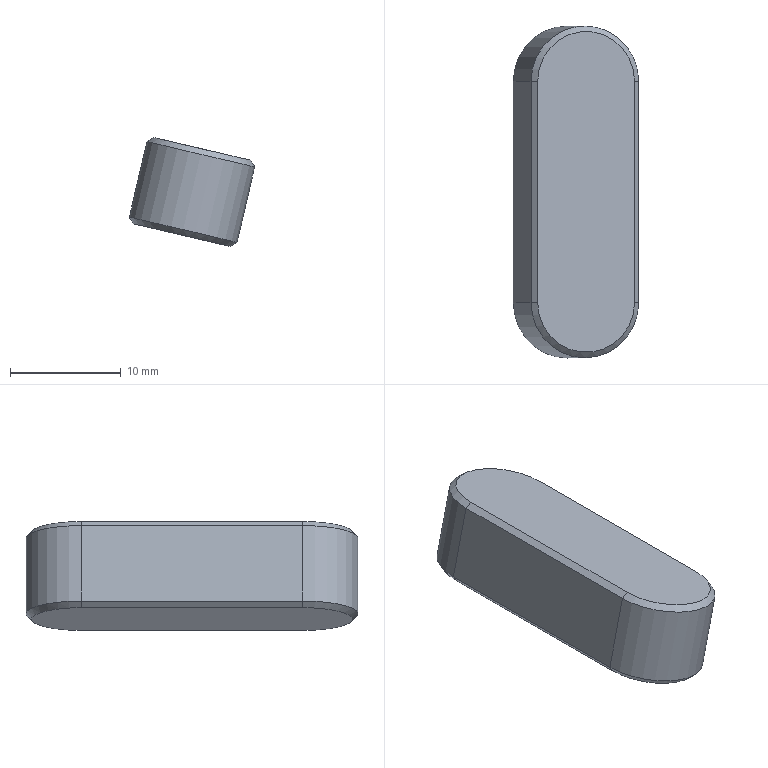Component | NX | SHAFT_KEY | 1 solid | 14 faces | box 11.34 x 30 x 9.85 mm | volume 2211 mm3 | plane 8 | cone 4 | cylinder 2 | commonest cylinder face diameters 10 x2
STEP:
#1=CARTESIAN_POINT('',(0.,0.,0.));
#2=DIRECTION('',(0.,0.,1.));
#3=DIRECTION('',(1.,0.,0.));
#4=AXIS2_PLACEMENT_3D('',#1,#2,#3);
#5=CARTESIAN_POINT('',(297.762,10.,102.339));
#6=VERTEX_POINT('',#5);
#7=CARTESIAN_POINT('',(299.362,10.,109.153));
#8=VERTEX_POINT('',#7);
#9=CARTESIAN_POINT('',(297.647,10.,101.852));
#10=DIRECTION('',(0.2286,0.,0.9735));
#11=VECTOR('',#10,1.);
#12=LINE('',#9,#11);
#13=CARTESIAN_POINT('',(302.515,10.,100.709));
#14=DIRECTION('',(0.2286,0.,0.9735));
#15=DIRECTION('',(0.,1.,0.));
#16=AXIS2_PLACEMENT_3D('',#13,#14,#15);
#17=CYLINDRICAL_SURFACE('',#16,5.);
#18=CARTESIAN_POINT('',(1.571,0.));
#19=DIRECTION('',(0.,1.));
#20=VECTOR('',#19,1.);
#21=LINE('',#18,#20);
#22=(GEOMETRIC_REPRESENTATION_CONTEXT(2)PARAMETRIC_REPRESENTATION_CONTEXT()REPRESENTATION_CONTEXT('',''));
#23=DEFINITIONAL_REPRESENTATION('',(#21),#22);
#24=PCURVE('',#17,#23);
#25=CARTESIAN_POINT('',(297.647,-10.,101.852));
#26=DIRECTION('',(0.9735,0.,-0.2286));
#27=DIRECTION('',(0.2286,0.,0.9735));
#28=AXIS2_PLACEMENT_3D('',#25,#26,#27);
#29=PLANE('',#28);
#30=CARTESIAN_POINT('',(0.,-20.));
#31=DIRECTION('',(1.,0.));
#32=VECTOR('',#31,1.);
#33=LINE('',#30,#32);
#34=(GEOMETRIC_REPRESENTATION_CONTEXT(2)PARAMETRIC_REPRESENTATION_CONTEXT()REPRESENTATION_CONTEXT('',''));
#35=DEFINITIONAL_REPRESENTATION('',(#33),#34);
#36=PCURVE('',#29,#35);
#37=SURFACE_CURVE('',#12,(#24,#36),.PCURVE_S1.);
#38=EDGE_CURVE('',#6,#8,#37,.T.);
#39=ORIENTED_EDGE('',*,*,#38,.T.);
#40=CARTESIAN_POINT('',(309.097,10.,106.867));
#41=VERTEX_POINT('',#40);
#42=CARTESIAN_POINT('',(304.229,10.,108.01));
#43=DIRECTION('',(-0.2286,0.,-0.9735));
#44=DIRECTION('',(0.,-1.,0.));
#45=AXIS2_PLACEMENT_3D('',#42,#43,#44);
#46=CIRCLE('',#45,5.);
#47=CARTESIAN_POINT('',(3.142,7.5));
#48=DIRECTION('',(-1.,0.));
#49=VECTOR('',#48,1.);
#50=LINE('',#47,#49);
#51=(GEOMETRIC_REPRESENTATION_CONTEXT(2)PARAMETRIC_REPRESENTATION_CONTEXT()REPRESENTATION_CONTEXT('',''));
#52=DEFINITIONAL_REPRESENTATION('',(#50),#51);
#53=PCURVE('',#17,#52);
#54=CARTESIAN_POINT('',(304.229,10.,108.01));
#55=DIRECTION('',(-0.2286,0.,-0.9735));
#56=DIRECTION('',(0.,-1.,-0.));
#57=AXIS2_PLACEMENT_3D('',#54,#55,#56);
#58=CONICAL_SURFACE('',#57,5.,0.7854);
#59=CARTESIAN_POINT('',(0.,0.));
#60=DIRECTION('',(1.,0.));
#61=VECTOR('',#60,1.);
#62=LINE('',#59,#61);
#63=(GEOMETRIC_REPRESENTATION_CONTEXT(2)PARAMETRIC_REPRESENTATION_CONTEXT()REPRESENTATION_CONTEXT('',''));
#64=DEFINITIONAL_REPRESENTATION('',(#62),#63);
#65=PCURVE('',#58,#64);
#66=SURFACE_CURVE('',#46,(#53,#65),.PCURVE_S1.);
#67=EDGE_CURVE('',#8,#41,#66,.T.);
#68=ORIENTED_EDGE('',*,*,#67,.T.);
#69=CARTESIAN_POINT('',(307.497,10.,100.052));
#70=VERTEX_POINT('',#69);
#71=CARTESIAN_POINT('',(307.382,10.,99.566));
#72=DIRECTION('',(0.2286,0.,0.9735));
#73=VECTOR('',#72,1.);
#74=LINE('',#71,#73);
#75=CARTESIAN_POINT('',(-1.571,-0.));
#76=DIRECTION('',(0.,1.));
#77=VECTOR('',#76,1.);
#78=LINE('',#75,#77);
#79=(GEOMETRIC_REPRESENTATION_CONTEXT(2)PARAMETRIC_REPRESENTATION_CONTEXT()REPRESENTATION_CONTEXT('',''));
#80=DEFINITIONAL_REPRESENTATION('',(#78),#79);
#81=PCURVE('',#17,#80);
#82=CARTESIAN_POINT('',(307.382,10.,99.566));
#83=DIRECTION('',(-0.9735,0.,0.2286));
#84=DIRECTION('',(-0.2286,0.,-0.9735));
#85=AXIS2_PLACEMENT_3D('',#82,#83,#84);
#86=PLANE('',#85);
#87=CARTESIAN_POINT('',(0.,0.));
#88=DIRECTION('',(-1.,0.));
#89=VECTOR('',#88,1.);
#90=LINE('',#87,#89);
#91=(GEOMETRIC_REPRESENTATION_CONTEXT(2)PARAMETRIC_REPRESENTATION_CONTEXT()REPRESENTATION_CONTEXT('',''));
#92=DEFINITIONAL_REPRESENTATION('',(#90),#91);
#93=PCURVE('',#86,#92);
#94=SURFACE_CURVE('',#74,(#81,#93),.PCURVE_S1.);
#95=EDGE_CURVE('',#70,#41,#94,.T.);
#96=ORIENTED_EDGE('',*,*,#95,.F.);
#97=CARTESIAN_POINT('',(302.629,10.,101.195));
#98=DIRECTION('',(0.2286,0.,0.9735));
#99=DIRECTION('',(0.,-1.,0.));
#100=AXIS2_PLACEMENT_3D('',#97,#98,#99);
#101=CIRCLE('',#100,5.);
#102=CARTESIAN_POINT('',(-3.142,0.5));
#103=DIRECTION('',(1.,0.));
#104=VECTOR('',#103,1.);
#105=LINE('',#102,#104);
#106=(GEOMETRIC_REPRESENTATION_CONTEXT(2)PARAMETRIC_REPRESENTATION_CONTEXT()REPRESENTATION_CONTEXT('',''));
#107=DEFINITIONAL_REPRESENTATION('',(#105),#106);
#108=PCURVE('',#17,#107);
#109=CARTESIAN_POINT('',(302.515,10.,100.709));
#110=DIRECTION('',(0.2286,0.,0.9735));
#111=DIRECTION('',(0.,1.,-0.));
#112=AXIS2_PLACEMENT_3D('',#109,#110,#111);
#113=CONICAL_SURFACE('',#112,4.5,0.7854);
#114=CARTESIAN_POINT('',(-3.142,0.5));
#115=DIRECTION('',(1.,0.));
#116=VECTOR('',#115,1.);
#117=LINE('',#114,#116);
#118=(GEOMETRIC_REPRESENTATION_CONTEXT(2)PARAMETRIC_REPRESENTATION_CONTEXT()REPRESENTATION_CONTEXT('',''));
#119=DEFINITIONAL_REPRESENTATION('',(#117),#118);
#120=PCURVE('',#113,#119);
#121=SURFACE_CURVE('',#101,(#108,#120),.PCURVE_S1.);
#122=EDGE_CURVE('',#70,#6,#121,.T.);
#123=ORIENTED_EDGE('',*,*,#122,.T.);
#124=EDGE_LOOP('',(#39,#68,#96,#123));
#125=FACE_BOUND('',#124,.T.);
#126=ADVANCED_FACE('',(#125),#17,.T.);
#127=ORIENTED_EDGE('',*,*,#95,.T.);
#128=CARTESIAN_POINT('',(309.097,-10.,106.867));
#129=VERTEX_POINT('',#128);
#130=CARTESIAN_POINT('',(309.097,10.,106.867));
#131=DIRECTION('',(0.,-1.,0.));
#132=VECTOR('',#131,1.);
#133=LINE('',#130,#132);
#134=CARTESIAN_POINT('',(-7.5,0.));
#135=DIRECTION('',(0.,1.));
#136=VECTOR('',#135,1.);
#137=LINE('',#134,#136);
#138=(GEOMETRIC_REPRESENTATION_CONTEXT(2)PARAMETRIC_REPRESENTATION_CONTEXT()REPRESENTATION_CONTEXT('',''));
#139=DEFINITIONAL_REPRESENTATION('',(#137),#138);
#140=PCURVE('',#86,#139);
#141=CARTESIAN_POINT('',(309.097,10.,106.867));
#142=DIRECTION('',(-0.85,0.,-0.5267));
#143=DIRECTION('',(0.,-1.,0.));
#144=AXIS2_PLACEMENT_3D('',#141,#142,#143);
#145=PLANE('',#144);
#146=CARTESIAN_POINT('',(0.,0.));
#147=DIRECTION('',(1.,0.));
#148=VECTOR('',#147,1.);
#149=LINE('',#146,#148);
#150=(GEOMETRIC_REPRESENTATION_CONTEXT(2)PARAMETRIC_REPRESENTATION_CONTEXT()REPRESENTATION_CONTEXT('',''));
#151=DEFINITIONAL_REPRESENTATION('',(#149),#150);
#152=PCURVE('',#145,#151);
#153=SURFACE_CURVE('',#133,(#140,#152),.PCURVE_S1.);
#154=EDGE_CURVE('',#41,#129,#153,.T.);
#155=ORIENTED_EDGE('',*,*,#154,.T.);
#156=CARTESIAN_POINT('',(307.497,-10.,100.052));
#157=VERTEX_POINT('',#156);
#158=CARTESIAN_POINT('',(307.382,-10.,99.566));
#159=DIRECTION('',(0.2286,0.,0.9735));
#160=VECTOR('',#159,1.);
#161=LINE('',#158,#160);
#162=CARTESIAN_POINT('',(0.,20.));
#163=DIRECTION('',(-1.,0.));
#164=VECTOR('',#163,1.);
#165=LINE('',#162,#164);
#166=(GEOMETRIC_REPRESENTATION_CONTEXT(2)PARAMETRIC_REPRESENTATION_CONTEXT()REPRESENTATION_CONTEXT('',''));
#167=DEFINITIONAL_REPRESENTATION('',(#165),#166);
#168=PCURVE('',#86,#167);
#169=CARTESIAN_POINT('',(302.515,-10.,100.709));
#170=DIRECTION('',(0.2286,0.,0.9735));
#171=DIRECTION('',(0.,1.,0.));
#172=AXIS2_PLACEMENT_3D('',#169,#170,#171);
#173=CYLINDRICAL_SURFACE('',#172,5.);
#174=CARTESIAN_POINT('',(4.712,-0.));
#175=DIRECTION('',(0.,1.));
#176=VECTOR('',#175,1.);
#177=LINE('',#174,#176);
#178=(GEOMETRIC_REPRESENTATION_CONTEXT(2)PARAMETRIC_REPRESENTATION_CONTEXT()REPRESENTATION_CONTEXT('',''));
#179=DEFINITIONAL_REPRESENTATION('',(#177),#178);
#180=PCURVE('',#173,#179);
#181=SURFACE_CURVE('',#161,(#168,#180),.PCURVE_S1.);
#182=EDGE_CURVE('',#157,#129,#181,.T.);
#183=ORIENTED_EDGE('',*,*,#182,.F.);
#184=CARTESIAN_POINT('',(307.497,10.,100.052));
#185=DIRECTION('',(0.,1.,0.));
#186=VECTOR('',#185,1.);
#187=LINE('',#184,#186);
#188=CARTESIAN_POINT('',(-0.5,0.));
#189=DIRECTION('',(0.,-1.));
#190=VECTOR('',#189,1.);
#191=LINE('',#188,#190);
#192=(GEOMETRIC_REPRESENTATION_CONTEXT(2)PARAMETRIC_REPRESENTATION_CONTEXT()REPRESENTATION_CONTEXT('',''));
#193=DEFINITIONAL_REPRESENTATION('',(#191),#192);
#194=PCURVE('',#86,#193);
#195=CARTESIAN_POINT('',(306.896,10.,99.68));
#196=DIRECTION('',(0.5267,0.,-0.85));
#197=DIRECTION('',(0.,1.,0.));
#198=AXIS2_PLACEMENT_3D('',#195,#196,#197);
#199=PLANE('',#198);
#200=CARTESIAN_POINT('',(-0.,0.7071));
#201=DIRECTION('',(1.,0.));
#202=VECTOR('',#201,1.);
#203=LINE('',#200,#202);
#204=(GEOMETRIC_REPRESENTATION_CONTEXT(2)PARAMETRIC_REPRESENTATION_CONTEXT()REPRESENTATION_CONTEXT('',''));
#205=DEFINITIONAL_REPRESENTATION('',(#203),#204);
#206=PCURVE('',#199,#205);
#207=SURFACE_CURVE('',#187,(#194,#206),.PCURVE_S1.);
#208=EDGE_CURVE('',#157,#70,#207,.T.);
#209=ORIENTED_EDGE('',*,*,#208,.T.);
#210=EDGE_LOOP('',(#127,#155,#183,#209));
#211=FACE_BOUND('',#210,.T.);
#212=ADVANCED_FACE('',(#211),#86,.F.);
#213=ORIENTED_EDGE('',*,*,#182,.T.);
#214=CARTESIAN_POINT('',(299.362,-10.,109.153));
#215=VERTEX_POINT('',#214);
#216=CARTESIAN_POINT('',(304.229,-10.,108.01));
#217=DIRECTION('',(-0.2286,0.,-0.9735));
#218=DIRECTION('',(0.,-1.,0.));
#219=AXIS2_PLACEMENT_3D('',#216,#217,#218);
#220=CIRCLE('',#219,5.);
#221=CARTESIAN_POINT('',(9.425,7.5));
#222=DIRECTION('',(-1.,0.));
#223=VECTOR('',#222,1.);
#224=LINE('',#221,#223);
#225=(GEOMETRIC_REPRESENTATION_CONTEXT(2)PARAMETRIC_REPRESENTATION_CONTEXT()REPRESENTATION_CONTEXT('',''));
#226=DEFINITIONAL_REPRESENTATION('',(#224),#225);
#227=PCURVE('',#173,#226);
#228=CARTESIAN_POINT('',(304.229,-10.,108.01));
#229=DIRECTION('',(-0.2286,0.,-0.9735));
#230=DIRECTION('',(0.,-1.,-0.));
#231=AXIS2_PLACEMENT_3D('',#228,#229,#230);
#232=CONICAL_SURFACE('',#231,5.,0.7854);
#233=CARTESIAN_POINT('',(0.,0.));
#234=DIRECTION('',(1.,0.));
#235=VECTOR('',#234,1.);
#236=LINE('',#233,#235);
#237=(GEOMETRIC_REPRESENTATION_CONTEXT(2)PARAMETRIC_REPRESENTATION_CONTEXT()REPRESENTATION_CONTEXT('',''));
#238=DEFINITIONAL_REPRESENTATION('',(#236),#237);
#239=PCURVE('',#232,#238);
#240=SURFACE_CURVE('',#220,(#227,#239),.PCURVE_S1.);
#241=EDGE_CURVE('',#129,#215,#240,.T.);
#242=ORIENTED_EDGE('',*,*,#241,.T.);
#243=CARTESIAN_POINT('',(297.762,-10.,102.339));
#244=VERTEX_POINT('',#243);
#245=CARTESIAN_POINT('',(297.647,-10.,101.852));
#246=DIRECTION('',(0.2286,0.,0.9735));
#247=VECTOR('',#246,1.);
#248=LINE('',#245,#247);
#249=CARTESIAN_POINT('',(1.571,0.));
#250=DIRECTION('',(0.,1.));
#251=VECTOR('',#250,1.);
#252=LINE('',#249,#251);
#253=(GEOMETRIC_REPRESENTATION_CONTEXT(2)PARAMETRIC_REPRESENTATION_CONTEXT()REPRESENTATION_CONTEXT('',''));
#254=DEFINITIONAL_REPRESENTATION('',(#252),#253);
#255=PCURVE('',#173,#254);
#256=CARTESIAN_POINT('',(0.,0.));
#257=DIRECTION('',(1.,0.));
#258=VECTOR('',#257,1.);
#259=LINE('',#256,#258);
#260=(GEOMETRIC_REPRESENTATION_CONTEXT(2)PARAMETRIC_REPRESENTATION_CONTEXT()REPRESENTATION_CONTEXT('',''));
#261=DEFINITIONAL_REPRESENTATION('',(#259),#260);
#262=PCURVE('',#29,#261);
#263=SURFACE_CURVE('',#248,(#255,#262),.PCURVE_S1.);
#264=EDGE_CURVE('',#244,#215,#263,.T.);
#265=ORIENTED_EDGE('',*,*,#264,.F.);
#266=CARTESIAN_POINT('',(302.629,-10.,101.195));
#267=DIRECTION('',(0.2286,0.,0.9735));
#268=DIRECTION('',(0.,-1.,0.));
#269=AXIS2_PLACEMENT_3D('',#266,#267,#268);
#270=CIRCLE('',#269,5.);
#271=CARTESIAN_POINT('',(-3.142,0.5));
#272=DIRECTION('',(1.,0.));
#273=VECTOR('',#272,1.);
#274=LINE('',#271,#273);
#275=(GEOMETRIC_REPRESENTATION_CONTEXT(2)PARAMETRIC_REPRESENTATION_CONTEXT()REPRESENTATION_CONTEXT('',''));
#276=DEFINITIONAL_REPRESENTATION('',(#274),#275);
#277=PCURVE('',#173,#276);
#278=CARTESIAN_POINT('',(302.515,-10.,100.709));
#279=DIRECTION('',(0.2286,0.,0.9735));
#280=DIRECTION('',(0.,1.,-0.));
#281=AXIS2_PLACEMENT_3D('',#278,#279,#280);
#282=CONICAL_SURFACE('',#281,4.5,0.7854);
#283=CARTESIAN_POINT('',(-3.142,0.5));
#284=DIRECTION('',(1.,-0.));
#285=VECTOR('',#284,1.);
#286=LINE('',#283,#285);
#287=(GEOMETRIC_REPRESENTATION_CONTEXT(2)PARAMETRIC_REPRESENTATION_CONTEXT()REPRESENTATION_CONTEXT('',''));
#288=DEFINITIONAL_REPRESENTATION('',(#286),#287);
#289=PCURVE('',#282,#288);
#290=SURFACE_CURVE('',#270,(#277,#289),.PCURVE_S1.);
#291=EDGE_CURVE('',#244,#157,#290,.T.);
#292=ORIENTED_EDGE('',*,*,#291,.T.);
#293=EDGE_LOOP('',(#213,#242,#265,#292));
#294=FACE_BOUND('',#293,.T.);
#295=ADVANCED_FACE('',(#294),#173,.T.);
#296=ORIENTED_EDGE('',*,*,#264,.T.);
#297=CARTESIAN_POINT('',(299.362,-10.,109.153));
#298=DIRECTION('',(0.,1.,0.));
#299=VECTOR('',#298,1.);
#300=LINE('',#297,#299);
#301=CARTESIAN_POINT('',(7.5,0.));
#302=DIRECTION('',(0.,-1.));
#303=VECTOR('',#302,1.);
#304=LINE('',#301,#303);
#305=(GEOMETRIC_REPRESENTATION_CONTEXT(2)PARAMETRIC_REPRESENTATION_CONTEXT()REPRESENTATION_CONTEXT('',''));
#306=DEFINITIONAL_REPRESENTATION('',(#304),#305);
#307=PCURVE('',#29,#306);
#308=CARTESIAN_POINT('',(299.362,-10.,109.153));
#309=DIRECTION('',(0.5267,0.,-0.85));
#310=DIRECTION('',(0.,1.,0.));
#311=AXIS2_PLACEMENT_3D('',#308,#309,#310);
#312=PLANE('',#311);
#313=CARTESIAN_POINT('',(0.,0.));
#314=DIRECTION('',(1.,0.));
#315=VECTOR('',#314,1.);
#316=LINE('',#313,#315);
#317=(GEOMETRIC_REPRESENTATION_CONTEXT(2)PARAMETRIC_REPRESENTATION_CONTEXT()REPRESENTATION_CONTEXT('',''));
#318=DEFINITIONAL_REPRESENTATION('',(#316),#317);
#319=PCURVE('',#312,#318);
#320=SURFACE_CURVE('',#300,(#307,#319),.PCURVE_S1.);
#321=EDGE_CURVE('',#215,#8,#320,.T.);
#322=ORIENTED_EDGE('',*,*,#321,.T.);
#323=ORIENTED_EDGE('',*,*,#38,.F.);
#324=CARTESIAN_POINT('',(297.762,-10.,102.339));
#325=DIRECTION('',(0.,-1.,0.));
#326=VECTOR('',#325,1.);
#327=LINE('',#324,#326);
#328=CARTESIAN_POINT('',(0.5,0.));
#329=DIRECTION('',(0.,1.));
#330=VECTOR('',#329,1.);
#331=LINE('',#328,#330);
#332=(GEOMETRIC_REPRESENTATION_CONTEXT(2)PARAMETRIC_REPRESENTATION_CONTEXT()REPRESENTATION_CONTEXT('',''));
#333=DEFINITIONAL_REPRESENTATION('',(#331),#332);
#334=PCURVE('',#29,#333);
#335=CARTESIAN_POINT('',(298.134,10.,101.737));
#336=DIRECTION('',(-0.85,0.,-0.5267));
#337=DIRECTION('',(0.,-1.,0.));
#338=AXIS2_PLACEMENT_3D('',#335,#336,#337);
#339=PLANE('',#338);
#340=CARTESIAN_POINT('',(20.,0.7071));
#341=DIRECTION('',(1.,0.));
#342=VECTOR('',#341,1.);
#343=LINE('',#340,#342);
#344=(GEOMETRIC_REPRESENTATION_CONTEXT(2)PARAMETRIC_REPRESENTATION_CONTEXT()REPRESENTATION_CONTEXT('',''));
#345=DEFINITIONAL_REPRESENTATION('',(#343),#344);
#346=PCURVE('',#339,#345);
#347=SURFACE_CURVE('',#327,(#334,#346),.PCURVE_S1.);
#348=EDGE_CURVE('',#6,#244,#347,.T.);
#349=ORIENTED_EDGE('',*,*,#348,.T.);
#350=EDGE_LOOP('',(#296,#322,#323,#349));
#351=FACE_BOUND('',#350,.T.);
#352=ADVANCED_FACE('',(#351),#29,.F.);
#353=CARTESIAN_POINT('',(298.134,-10.,101.737));
#354=VERTEX_POINT('',#353);
#355=CARTESIAN_POINT('',(298.134,10.,101.737));
#356=VERTEX_POINT('',#355);
#357=CARTESIAN_POINT('',(298.134,10.,101.737));
#358=DIRECTION('',(0.,1.,0.));
#359=VECTOR('',#358,1.);
#360=LINE('',#357,#359);
#361=CARTESIAN_POINT('',(302.515,10.,100.709));
#362=DIRECTION('',(-0.2286,0.,-0.9735));
#363=DIRECTION('',(0.,-1.,0.));
#364=AXIS2_PLACEMENT_3D('',#361,#362,#363);
#365=PLANE('',#364);
#366=CARTESIAN_POINT('',(0.,4.5));
#367=DIRECTION('',(-1.,0.));
#368=VECTOR('',#367,1.);
#369=LINE('',#366,#368);
#370=(GEOMETRIC_REPRESENTATION_CONTEXT(2)PARAMETRIC_REPRESENTATION_CONTEXT()REPRESENTATION_CONTEXT('',''));
#371=DEFINITIONAL_REPRESENTATION('',(#369),#370);
#372=PCURVE('',#365,#371);
#373=CARTESIAN_POINT('',(0.,0.));
#374=DIRECTION('',(-1.,0.));
#375=VECTOR('',#374,1.);
#376=LINE('',#373,#375);
#377=(GEOMETRIC_REPRESENTATION_CONTEXT(2)PARAMETRIC_REPRESENTATION_CONTEXT()REPRESENTATION_CONTEXT('',''));
#378=DEFINITIONAL_REPRESENTATION('',(#376),#377);
#379=PCURVE('',#339,#378);
#380=SURFACE_CURVE('',#360,(#372,#379),.PCURVE_S1.);
#381=EDGE_CURVE('',#354,#356,#380,.T.);
#382=ORIENTED_EDGE('',*,*,#381,.T.);
#383=CARTESIAN_POINT('',(306.896,10.,99.68));
#384=VERTEX_POINT('',#383);
#385=CARTESIAN_POINT('',(302.515,10.,100.709));
#386=DIRECTION('',(-0.2286,0.,-0.9735));
#387=DIRECTION('',(0.,-1.,0.));
#388=AXIS2_PLACEMENT_3D('',#385,#386,#387);
#389=CIRCLE('',#388,4.5);
#390=CARTESIAN_POINT('',(0.,0.));
#391=DIRECTION('',(1.,0.));
#392=AXIS2_PLACEMENT_2D('',#390,#391);
#393=CIRCLE('',#392,4.5);
#394=(GEOMETRIC_REPRESENTATION_CONTEXT(2)PARAMETRIC_REPRESENTATION_CONTEXT()REPRESENTATION_CONTEXT('',''));
#395=DEFINITIONAL_REPRESENTATION('',(#393),#394);
#396=PCURVE('',#365,#395);
#397=CARTESIAN_POINT('',(3.142,0.));
#398=DIRECTION('',(-1.,-0.));
#399=VECTOR('',#398,1.);
#400=LINE('',#397,#399);
#401=(GEOMETRIC_REPRESENTATION_CONTEXT(2)PARAMETRIC_REPRESENTATION_CONTEXT()REPRESENTATION_CONTEXT('',''));
#402=DEFINITIONAL_REPRESENTATION('',(#400),#401);
#403=PCURVE('',#113,#402);
#404=SURFACE_CURVE('',#389,(#396,#403),.PCURVE_S1.);
#405=EDGE_CURVE('',#356,#384,#404,.T.);
#406=ORIENTED_EDGE('',*,*,#405,.T.);
#407=CARTESIAN_POINT('',(306.896,-10.,99.68));
#408=VERTEX_POINT('',#407);
#409=CARTESIAN_POINT('',(306.896,-10.,99.68));
#410=DIRECTION('',(0.,-1.,0.));
#411=VECTOR('',#410,1.);
#412=LINE('',#409,#411);
#413=CARTESIAN_POINT('',(20.,-4.5));
#414=DIRECTION('',(1.,0.));
#415=VECTOR('',#414,1.);
#416=LINE('',#413,#415);
#417=(GEOMETRIC_REPRESENTATION_CONTEXT(2)PARAMETRIC_REPRESENTATION_CONTEXT()REPRESENTATION_CONTEXT('',''));
#418=DEFINITIONAL_REPRESENTATION('',(#416),#417);
#419=PCURVE('',#365,#418);
#420=CARTESIAN_POINT('',(-20.,0.));
#421=DIRECTION('',(-1.,0.));
#422=VECTOR('',#421,1.);
#423=LINE('',#420,#422);
#424=(GEOMETRIC_REPRESENTATION_CONTEXT(2)PARAMETRIC_REPRESENTATION_CONTEXT()REPRESENTATION_CONTEXT('',''));
#425=DEFINITIONAL_REPRESENTATION('',(#423),#424);
#426=PCURVE('',#199,#425);
#427=SURFACE_CURVE('',#412,(#419,#426),.PCURVE_S1.);
#428=EDGE_CURVE('',#384,#408,#427,.T.);
#429=ORIENTED_EDGE('',*,*,#428,.T.);
#430=CARTESIAN_POINT('',(302.515,-10.,100.709));
#431=DIRECTION('',(-0.2286,0.,-0.9735));
#432=DIRECTION('',(0.,-1.,0.));
#433=AXIS2_PLACEMENT_3D('',#430,#431,#432);
#434=CIRCLE('',#433,4.5);
#435=CARTESIAN_POINT('',(20.,0.));
#436=DIRECTION('',(1.,0.));
#437=AXIS2_PLACEMENT_2D('',#435,#436);
#438=CIRCLE('',#437,4.5);
#439=(GEOMETRIC_REPRESENTATION_CONTEXT(2)PARAMETRIC_REPRESENTATION_CONTEXT()REPRESENTATION_CONTEXT('',''));
#440=DEFINITIONAL_REPRESENTATION('',(#438),#439);
#441=PCURVE('',#365,#440);
#442=CARTESIAN_POINT('',(9.425,-0.));
#443=DIRECTION('',(-1.,0.));
#444=VECTOR('',#443,1.);
#445=LINE('',#442,#444);
#446=(GEOMETRIC_REPRESENTATION_CONTEXT(2)PARAMETRIC_REPRESENTATION_CONTEXT()REPRESENTATION_CONTEXT('',''));
#447=DEFINITIONAL_REPRESENTATION('',(#445),#446);
#448=PCURVE('',#282,#447);
#449=SURFACE_CURVE('',#434,(#441,#448),.PCURVE_S1.);
#450=EDGE_CURVE('',#408,#354,#449,.T.);
#451=ORIENTED_EDGE('',*,*,#450,.T.);
#452=EDGE_LOOP('',(#382,#406,#429,#451));
#453=FACE_BOUND('',#452,.T.);
#454=ADVANCED_FACE('',(#453),#365,.T.);
#455=CARTESIAN_POINT('',(308.725,-10.,107.468));
#456=VERTEX_POINT('',#455);
#457=CARTESIAN_POINT('',(308.725,10.,107.468));
#458=VERTEX_POINT('',#457);
#459=CARTESIAN_POINT('',(308.725,10.,107.468));
#460=DIRECTION('',(0.,1.,0.));
#461=VECTOR('',#460,1.);
#462=LINE('',#459,#461);
#463=CARTESIAN_POINT('',(304.344,10.,108.497));
#464=DIRECTION('',(-0.2286,0.,-0.9735));
#465=DIRECTION('',(0.,-1.,0.));
#466=AXIS2_PLACEMENT_3D('',#463,#464,#465);
#467=PLANE('',#466);
#468=CARTESIAN_POINT('',(0.,-4.5));
#469=DIRECTION('',(-1.,0.));
#470=VECTOR('',#469,1.);
#471=LINE('',#468,#470);
#472=(GEOMETRIC_REPRESENTATION_CONTEXT(2)PARAMETRIC_REPRESENTATION_CONTEXT()REPRESENTATION_CONTEXT('',''));
#473=DEFINITIONAL_REPRESENTATION('',(#471),#472);
#474=PCURVE('',#467,#473);
#475=CARTESIAN_POINT('',(0.,0.7071));
#476=DIRECTION('',(-1.,0.));
#477=VECTOR('',#476,1.);
#478=LINE('',#475,#477);
#479=(GEOMETRIC_REPRESENTATION_CONTEXT(2)PARAMETRIC_REPRESENTATION_CONTEXT()REPRESENTATION_CONTEXT('',''));
#480=DEFINITIONAL_REPRESENTATION('',(#478),#479);
#481=PCURVE('',#145,#480);
#482=SURFACE_CURVE('',#462,(#474,#481),.PCURVE_S1.);
#483=EDGE_CURVE('',#456,#458,#482,.T.);
#484=ORIENTED_EDGE('',*,*,#483,.T.);
#485=CARTESIAN_POINT('',(299.963,10.,109.526));
#486=VERTEX_POINT('',#485);
#487=CARTESIAN_POINT('',(304.344,10.,108.497));
#488=DIRECTION('',(0.2286,0.,0.9735));
#489=DIRECTION('',(0.,-1.,0.));
#490=AXIS2_PLACEMENT_3D('',#487,#488,#489);
#491=CIRCLE('',#490,4.5);
#492=CARTESIAN_POINT('',(4.5,0.));
#493=CARTESIAN_POINT('',(4.5,-7.794));
#494=CARTESIAN_POINT('',(-2.25,-3.897));
#495=CARTESIAN_POINT('',(-9.,-0.));
#496=CARTESIAN_POINT('',(-2.25,3.897));
#497=CARTESIAN_POINT('',(4.5,7.794));
#498=CARTESIAN_POINT('',(4.5,0.));
#499=(BOUNDED_CURVE()B_SPLINE_CURVE(2,(#492,#493,#494,#495,#496,#497,#498),.UNSPECIFIED.,.T.,.F.)B_SPLINE_CURVE_WITH_KNOTS((1,2,2,2,2,1),(-2.094,0.,2.094,4.189,6.283,8.378),.UNSPECIFIED.)CURVE()GEOMETRIC_REPRESENTATION_ITEM()RATIONAL_B_SPLINE_CURVE((1.,0.5,1.,0.5,1.,0.5,1.))REPRESENTATION_ITEM(''));
#500=(GEOMETRIC_REPRESENTATION_CONTEXT(2)PARAMETRIC_REPRESENTATION_CONTEXT()REPRESENTATION_CONTEXT('',''));
#501=DEFINITIONAL_REPRESENTATION('',(#499),#500);
#502=PCURVE('',#467,#501);
#503=CARTESIAN_POINT('',(6.283,-0.5));
#504=DIRECTION('',(-1.,-0.));
#505=VECTOR('',#504,1.);
#506=LINE('',#503,#505);
#507=(GEOMETRIC_REPRESENTATION_CONTEXT(2)PARAMETRIC_REPRESENTATION_CONTEXT()REPRESENTATION_CONTEXT('',''));
#508=DEFINITIONAL_REPRESENTATION('',(#506),#507);
#509=PCURVE('',#58,#508);
#510=SURFACE_CURVE('',#491,(#502,#509),.PCURVE_S1.);
#511=EDGE_CURVE('',#458,#486,#510,.T.);
#512=ORIENTED_EDGE('',*,*,#511,.T.);
#513=CARTESIAN_POINT('',(299.963,-10.,109.526));
#514=VERTEX_POINT('',#513);
#515=CARTESIAN_POINT('',(299.963,10.,109.526));
#516=DIRECTION('',(0.,-1.,0.));
#517=VECTOR('',#516,1.);
#518=LINE('',#515,#517);
#519=CARTESIAN_POINT('',(0.,4.5));
#520=DIRECTION('',(1.,0.));
#521=VECTOR('',#520,1.);
#522=LINE('',#519,#521);
#523=(GEOMETRIC_REPRESENTATION_CONTEXT(2)PARAMETRIC_REPRESENTATION_CONTEXT()REPRESENTATION_CONTEXT('',''));
#524=DEFINITIONAL_REPRESENTATION('',(#522),#523);
#525=PCURVE('',#467,#524);
#526=CARTESIAN_POINT('',(20.,0.7071));
#527=DIRECTION('',(-1.,0.));
#528=VECTOR('',#527,1.);
#529=LINE('',#526,#528);
#530=(GEOMETRIC_REPRESENTATION_CONTEXT(2)PARAMETRIC_REPRESENTATION_CONTEXT()REPRESENTATION_CONTEXT('',''));
#531=DEFINITIONAL_REPRESENTATION('',(#529),#530);
#532=PCURVE('',#312,#531);
#533=SURFACE_CURVE('',#518,(#525,#532),.PCURVE_S1.);
#534=EDGE_CURVE('',#486,#514,#533,.T.);
#535=ORIENTED_EDGE('',*,*,#534,.T.);
#536=CARTESIAN_POINT('',(304.344,-10.,108.497));
#537=DIRECTION('',(0.2286,0.,0.9735));
#538=DIRECTION('',(0.,-1.,0.));
#539=AXIS2_PLACEMENT_3D('',#536,#537,#538);
#540=CIRCLE('',#539,4.5);
#541=CARTESIAN_POINT('',(24.5,0.));
#542=CARTESIAN_POINT('',(24.5,-7.794));
#543=CARTESIAN_POINT('',(17.75,-3.897));
#544=CARTESIAN_POINT('',(11.,-0.));
#545=CARTESIAN_POINT('',(17.75,3.897));
#546=CARTESIAN_POINT('',(24.5,7.794));
#547=CARTESIAN_POINT('',(24.5,0.));
#548=(BOUNDED_CURVE()B_SPLINE_CURVE(2,(#541,#542,#543,#544,#545,#546,#547),.UNSPECIFIED.,.T.,.F.)B_SPLINE_CURVE_WITH_KNOTS((1,2,2,2,2,1),(-2.094,0.,2.094,4.189,6.283,8.378),.UNSPECIFIED.)CURVE()GEOMETRIC_REPRESENTATION_ITEM()RATIONAL_B_SPLINE_CURVE((1.,0.5,1.,0.5,1.,0.5,1.))REPRESENTATION_ITEM(''));
#549=(GEOMETRIC_REPRESENTATION_CONTEXT(2)PARAMETRIC_REPRESENTATION_CONTEXT()REPRESENTATION_CONTEXT('',''));
#550=DEFINITIONAL_REPRESENTATION('',(#548),#549);
#551=PCURVE('',#467,#550);
#552=CARTESIAN_POINT('',(12.566,-0.5));
#553=DIRECTION('',(-1.,0.));
#554=VECTOR('',#553,1.);
#555=LINE('',#552,#554);
#556=(GEOMETRIC_REPRESENTATION_CONTEXT(2)PARAMETRIC_REPRESENTATION_CONTEXT()REPRESENTATION_CONTEXT('',''));
#557=DEFINITIONAL_REPRESENTATION('',(#555),#556);
#558=PCURVE('',#232,#557);
#559=SURFACE_CURVE('',#540,(#551,#558),.PCURVE_S1.);
#560=EDGE_CURVE('',#514,#456,#559,.T.);
#561=ORIENTED_EDGE('',*,*,#560,.T.);
#562=EDGE_LOOP('',(#484,#512,#535,#561));
#563=FACE_BOUND('',#562,.T.);
#564=ADVANCED_FACE('',(#563),#467,.F.);
#565=CARTESIAN_POINT('',(308.725,-10.,107.468));
#566=DIRECTION('',(0.5267,0.,-0.85));
#567=VECTOR('',#566,1.);
#568=LINE('',#565,#567);
#569=CARTESIAN_POINT('',(4.712,-0.5));
#570=DIRECTION('',(0.,1.));
#571=VECTOR('',#570,1.);
#572=LINE('',#569,#571);
#573=(GEOMETRIC_REPRESENTATION_CONTEXT(2)PARAMETRIC_REPRESENTATION_CONTEXT()REPRESENTATION_CONTEXT('',''));
#574=DEFINITIONAL_REPRESENTATION('',(#572),#573);
#575=PCURVE('',#232,#574);
#576=CARTESIAN_POINT('',(20.,0.7071));
#577=DIRECTION('',(0.,-1.));
#578=VECTOR('',#577,1.);
#579=LINE('',#576,#578);
#580=(GEOMETRIC_REPRESENTATION_CONTEXT(2)PARAMETRIC_REPRESENTATION_CONTEXT()REPRESENTATION_CONTEXT('',''));
#581=DEFINITIONAL_REPRESENTATION('',(#579),#580);
#582=PCURVE('',#145,#581);
#583=SURFACE_CURVE('',#568,(#575,#582),.PCURVE_S1.);
#584=EDGE_CURVE('',#456,#129,#583,.T.);
#585=ORIENTED_EDGE('',*,*,#584,.F.);
#586=ORIENTED_EDGE('',*,*,#560,.F.);
#587=CARTESIAN_POINT('',(299.362,-10.,109.153));
#588=DIRECTION('',(0.85,0.,0.5267));
#589=VECTOR('',#588,1.);
#590=LINE('',#587,#589);
#591=CARTESIAN_POINT('',(7.854,-0.));
#592=DIRECTION('',(-0.,-1.));
#593=VECTOR('',#592,1.);
#594=LINE('',#591,#593);
#595=(GEOMETRIC_REPRESENTATION_CONTEXT(2)PARAMETRIC_REPRESENTATION_CONTEXT()REPRESENTATION_CONTEXT('',''));
#596=DEFINITIONAL_REPRESENTATION('',(#594),#595);
#597=PCURVE('',#232,#596);
#598=CARTESIAN_POINT('',(-0.,0.));
#599=DIRECTION('',(0.,1.));
#600=VECTOR('',#599,1.);
#601=LINE('',#598,#600);
#602=(GEOMETRIC_REPRESENTATION_CONTEXT(2)PARAMETRIC_REPRESENTATION_CONTEXT()REPRESENTATION_CONTEXT('',''));
#603=DEFINITIONAL_REPRESENTATION('',(#601),#602);
#604=PCURVE('',#312,#603);
#605=SURFACE_CURVE('',#590,(#597,#604),.PCURVE_S1.);
#606=EDGE_CURVE('',#215,#514,#605,.T.);
#607=ORIENTED_EDGE('',*,*,#606,.F.);
#608=ORIENTED_EDGE('',*,*,#241,.F.);
#609=EDGE_LOOP('',(#585,#586,#607,#608));
#610=FACE_BOUND('',#609,.T.);
#611=ADVANCED_FACE('',(#610),#232,.T.);
#612=ORIENTED_EDGE('',*,*,#606,.T.);
#613=ORIENTED_EDGE('',*,*,#534,.F.);
#614=CARTESIAN_POINT('',(299.362,10.,109.153));
#615=DIRECTION('',(0.85,0.,0.5267));
#616=VECTOR('',#615,1.);
#617=LINE('',#614,#616);
#618=CARTESIAN_POINT('',(20.,0.));
#619=DIRECTION('',(0.,1.));
#620=VECTOR('',#619,1.);
#621=LINE('',#618,#620);
#622=(GEOMETRIC_REPRESENTATION_CONTEXT(2)PARAMETRIC_REPRESENTATION_CONTEXT()REPRESENTATION_CONTEXT('',''));
#623=DEFINITIONAL_REPRESENTATION('',(#621),#622);
#624=PCURVE('',#312,#623);
#625=CARTESIAN_POINT('',(1.571,-0.));
#626=DIRECTION('',(0.,-1.));
#627=VECTOR('',#626,1.);
#628=LINE('',#625,#627);
#629=(GEOMETRIC_REPRESENTATION_CONTEXT(2)PARAMETRIC_REPRESENTATION_CONTEXT()REPRESENTATION_CONTEXT('',''));
#630=DEFINITIONAL_REPRESENTATION('',(#628),#629);
#631=PCURVE('',#58,#630);
#632=SURFACE_CURVE('',#617,(#624,#631),.PCURVE_S1.);
#633=EDGE_CURVE('',#8,#486,#632,.T.);
#634=ORIENTED_EDGE('',*,*,#633,.F.);
#635=ORIENTED_EDGE('',*,*,#321,.F.);
#636=EDGE_LOOP('',(#612,#613,#634,#635));
#637=FACE_BOUND('',#636,.T.);
#638=ADVANCED_FACE('',(#637),#312,.F.);
#639=ORIENTED_EDGE('',*,*,#584,.T.);
#640=ORIENTED_EDGE('',*,*,#154,.F.);
#641=CARTESIAN_POINT('',(308.725,10.,107.468));
#642=DIRECTION('',(0.5267,-0.,-0.85));
#643=VECTOR('',#642,1.);
#644=LINE('',#641,#643);
#645=CARTESIAN_POINT('',(0.,0.7071));
#646=DIRECTION('',(0.,-1.));
#647=VECTOR('',#646,1.);
#648=LINE('',#645,#647);
#649=(GEOMETRIC_REPRESENTATION_CONTEXT(2)PARAMETRIC_REPRESENTATION_CONTEXT()REPRESENTATION_CONTEXT('',''));
#650=DEFINITIONAL_REPRESENTATION('',(#648),#649);
#651=PCURVE('',#145,#650);
#652=CARTESIAN_POINT('',(4.712,-0.5));
#653=DIRECTION('',(0.,1.));
#654=VECTOR('',#653,1.);
#655=LINE('',#652,#654);
#656=(GEOMETRIC_REPRESENTATION_CONTEXT(2)PARAMETRIC_REPRESENTATION_CONTEXT()REPRESENTATION_CONTEXT('',''));
#657=DEFINITIONAL_REPRESENTATION('',(#655),#656);
#658=PCURVE('',#58,#657);
#659=SURFACE_CURVE('',#644,(#651,#658),.PCURVE_S1.);
#660=EDGE_CURVE('',#458,#41,#659,.T.);
#661=ORIENTED_EDGE('',*,*,#660,.F.);
#662=ORIENTED_EDGE('',*,*,#483,.F.);
#663=EDGE_LOOP('',(#639,#640,#661,#662));
#664=FACE_BOUND('',#663,.T.);
#665=ADVANCED_FACE('',(#664),#145,.F.);
#666=ORIENTED_EDGE('',*,*,#633,.T.);
#667=ORIENTED_EDGE('',*,*,#511,.F.);
#668=ORIENTED_EDGE('',*,*,#660,.T.);
#669=ORIENTED_EDGE('',*,*,#67,.F.);
#670=EDGE_LOOP('',(#666,#667,#668,#669));
#671=FACE_BOUND('',#670,.T.);
#672=ADVANCED_FACE('',(#671),#58,.T.);
#673=CARTESIAN_POINT('',(307.497,-10.,100.052));
#674=DIRECTION('',(-0.85,0.,-0.5267));
#675=VECTOR('',#674,1.);
#676=LINE('',#673,#675);
#677=CARTESIAN_POINT('',(4.712,0.5));
#678=DIRECTION('',(0.,-1.));
#679=VECTOR('',#678,1.);
#680=LINE('',#677,#679);
#681=(GEOMETRIC_REPRESENTATION_CONTEXT(2)PARAMETRIC_REPRESENTATION_CONTEXT()REPRESENTATION_CONTEXT('',''));
#682=DEFINITIONAL_REPRESENTATION('',(#680),#681);
#683=PCURVE('',#282,#682);
#684=CARTESIAN_POINT('',(-20.,0.7071));
#685=DIRECTION('',(0.,-1.));
#686=VECTOR('',#685,1.);
#687=LINE('',#684,#686);
#688=(GEOMETRIC_REPRESENTATION_CONTEXT(2)PARAMETRIC_REPRESENTATION_CONTEXT()REPRESENTATION_CONTEXT('',''));
#689=DEFINITIONAL_REPRESENTATION('',(#687),#688);
#690=PCURVE('',#199,#689);
#691=SURFACE_CURVE('',#676,(#683,#690),.PCURVE_S1.);
#692=EDGE_CURVE('',#157,#408,#691,.T.);
#693=ORIENTED_EDGE('',*,*,#692,.F.);
#694=ORIENTED_EDGE('',*,*,#291,.F.);
#695=CARTESIAN_POINT('',(298.134,-10.,101.737));
#696=DIRECTION('',(-0.5267,0.,0.85));
#697=VECTOR('',#696,1.);
#698=LINE('',#695,#697);
#699=CARTESIAN_POINT('',(1.571,-0.));
#700=DIRECTION('',(-0.,1.));
#701=VECTOR('',#700,1.);
#702=LINE('',#699,#701);
#703=(GEOMETRIC_REPRESENTATION_CONTEXT(2)PARAMETRIC_REPRESENTATION_CONTEXT()REPRESENTATION_CONTEXT('',''));
#704=DEFINITIONAL_REPRESENTATION('',(#702),#703);
#705=PCURVE('',#282,#704);
#706=CARTESIAN_POINT('',(20.,0.));
#707=DIRECTION('',(0.,1.));
#708=VECTOR('',#707,1.);
#709=LINE('',#706,#708);
#710=(GEOMETRIC_REPRESENTATION_CONTEXT(2)PARAMETRIC_REPRESENTATION_CONTEXT()REPRESENTATION_CONTEXT('',''));
#711=DEFINITIONAL_REPRESENTATION('',(#709),#710);
#712=PCURVE('',#339,#711);
#713=SURFACE_CURVE('',#698,(#705,#712),.PCURVE_S1.);
#714=EDGE_CURVE('',#354,#244,#713,.T.);
#715=ORIENTED_EDGE('',*,*,#714,.F.);
#716=ORIENTED_EDGE('',*,*,#450,.F.);
#717=EDGE_LOOP('',(#693,#694,#715,#716));
#718=FACE_BOUND('',#717,.T.);
#719=ADVANCED_FACE('',(#718),#282,.T.);
#720=ORIENTED_EDGE('',*,*,#714,.T.);
#721=ORIENTED_EDGE('',*,*,#348,.F.);
#722=CARTESIAN_POINT('',(298.134,10.,101.737));
#723=DIRECTION('',(-0.5267,-0.,0.85));
#724=VECTOR('',#723,1.);
#725=LINE('',#722,#724);
#726=CARTESIAN_POINT('',(0.,0.));
#727=DIRECTION('',(0.,1.));
#728=VECTOR('',#727,1.);
#729=LINE('',#726,#728);
#730=(GEOMETRIC_REPRESENTATION_CONTEXT(2)PARAMETRIC_REPRESENTATION_CONTEXT()REPRESENTATION_CONTEXT('',''));
#731=DEFINITIONAL_REPRESENTATION('',(#729),#730);
#732=PCURVE('',#339,#731);
#733=CARTESIAN_POINT('',(1.571,-0.));
#734=DIRECTION('',(0.,1.));
#735=VECTOR('',#734,1.);
#736=LINE('',#733,#735);
#737=(GEOMETRIC_REPRESENTATION_CONTEXT(2)PARAMETRIC_REPRESENTATION_CONTEXT()REPRESENTATION_CONTEXT('',''));
#738=DEFINITIONAL_REPRESENTATION('',(#736),#737);
#739=PCURVE('',#113,#738);
#740=SURFACE_CURVE('',#725,(#732,#739),.PCURVE_S1.);
#741=EDGE_CURVE('',#356,#6,#740,.T.);
#742=ORIENTED_EDGE('',*,*,#741,.F.);
#743=ORIENTED_EDGE('',*,*,#381,.F.);
#744=EDGE_LOOP('',(#720,#721,#742,#743));
#745=FACE_BOUND('',#744,.T.);
#746=ADVANCED_FACE('',(#745),#339,.T.);
#747=ORIENTED_EDGE('',*,*,#692,.T.);
#748=ORIENTED_EDGE('',*,*,#428,.F.);
#749=CARTESIAN_POINT('',(307.497,10.,100.052));
#750=DIRECTION('',(-0.85,0.,-0.5267));
#751=VECTOR('',#750,1.);
#752=LINE('',#749,#751);
#753=CARTESIAN_POINT('',(-0.,0.7071));
#754=DIRECTION('',(0.,-1.));
#755=VECTOR('',#754,1.);
#756=LINE('',#753,#755);
#757=(GEOMETRIC_REPRESENTATION_CONTEXT(2)PARAMETRIC_REPRESENTATION_CONTEXT()REPRESENTATION_CONTEXT('',''));
#758=DEFINITIONAL_REPRESENTATION('',(#756),#757);
#759=PCURVE('',#199,#758);
#760=CARTESIAN_POINT('',(-1.571,0.5));
#761=DIRECTION('',(0.,-1.));
#762=VECTOR('',#761,1.);
#763=LINE('',#760,#762);
#764=(GEOMETRIC_REPRESENTATION_CONTEXT(2)PARAMETRIC_REPRESENTATION_CONTEXT()REPRESENTATION_CONTEXT('',''));
#765=DEFINITIONAL_REPRESENTATION('',(#763),#764);
#766=PCURVE('',#113,#765);
#767=SURFACE_CURVE('',#752,(#759,#766),.PCURVE_S1.);
#768=EDGE_CURVE('',#70,#384,#767,.T.);
#769=ORIENTED_EDGE('',*,*,#768,.F.);
#770=ORIENTED_EDGE('',*,*,#208,.F.);
#771=EDGE_LOOP('',(#747,#748,#769,#770));
#772=FACE_BOUND('',#771,.T.);
#773=ADVANCED_FACE('',(#772),#199,.T.);
#774=ORIENTED_EDGE('',*,*,#741,.T.);
#775=ORIENTED_EDGE('',*,*,#122,.F.);
#776=ORIENTED_EDGE('',*,*,#768,.T.);
#777=ORIENTED_EDGE('',*,*,#405,.F.);
#778=EDGE_LOOP('',(#774,#775,#776,#777));
#779=FACE_BOUND('',#778,.T.);
#780=ADVANCED_FACE('',(#779),#113,.T.);
#781=CLOSED_SHELL('',(#126,#212,#295,#352,#454,#564,#611,#638,#665,#672,#719,#746,#773,#780));
#782=MANIFOLD_SOLID_BREP('',#781);
#783=(LENGTH_UNIT()NAMED_UNIT(*)SI_UNIT(.MILLI.,.METRE.));
#784=UNCERTAINTY_MEASURE_WITH_UNIT(LENGTH_MEASURE(0.0000001),#783,'','');
#785=(NAMED_UNIT(*)PLANE_ANGLE_UNIT()SI_UNIT($,.RADIAN.));
#786=(NAMED_UNIT(*)SI_UNIT($,.STERADIAN.)SOLID_ANGLE_UNIT());
#787=(GEOMETRIC_REPRESENTATION_CONTEXT(3)GLOBAL_UNCERTAINTY_ASSIGNED_CONTEXT((#784))GLOBAL_UNIT_ASSIGNED_CONTEXT((#783,#785,#786))REPRESENTATION_CONTEXT('',''));
#788=ADVANCED_BREP_SHAPE_REPRESENTATION('',(#4,#782),#787);